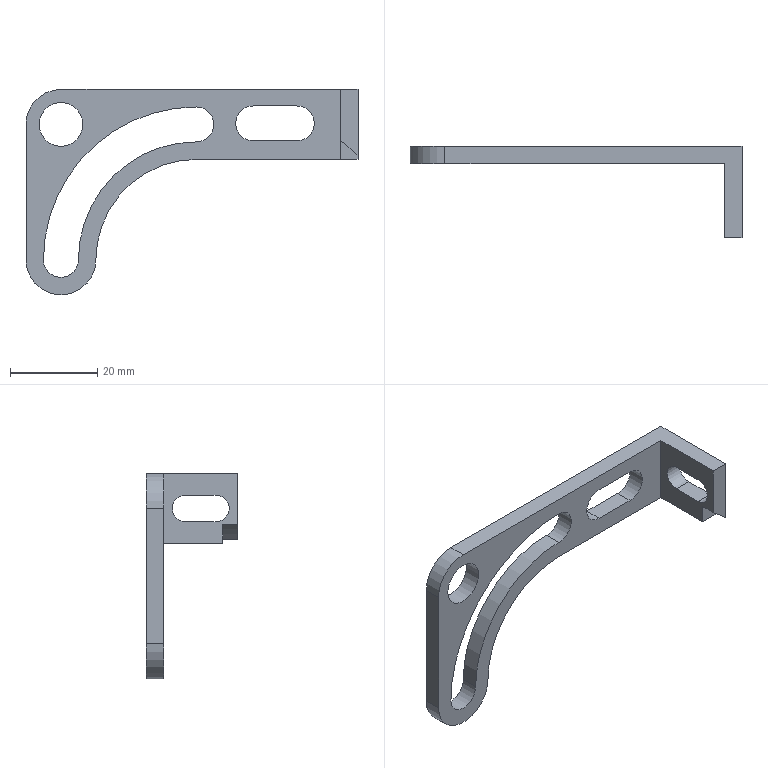Component | NX | MODEL5 | 1 solid | 26 faces | volume 5312 mm3 | cylinder 13 | plane 13 | commonest cylinder face diameters 8 x4 16 x2 6 x2 54 x1 46 x1 10 x1 70 x1 68 x1